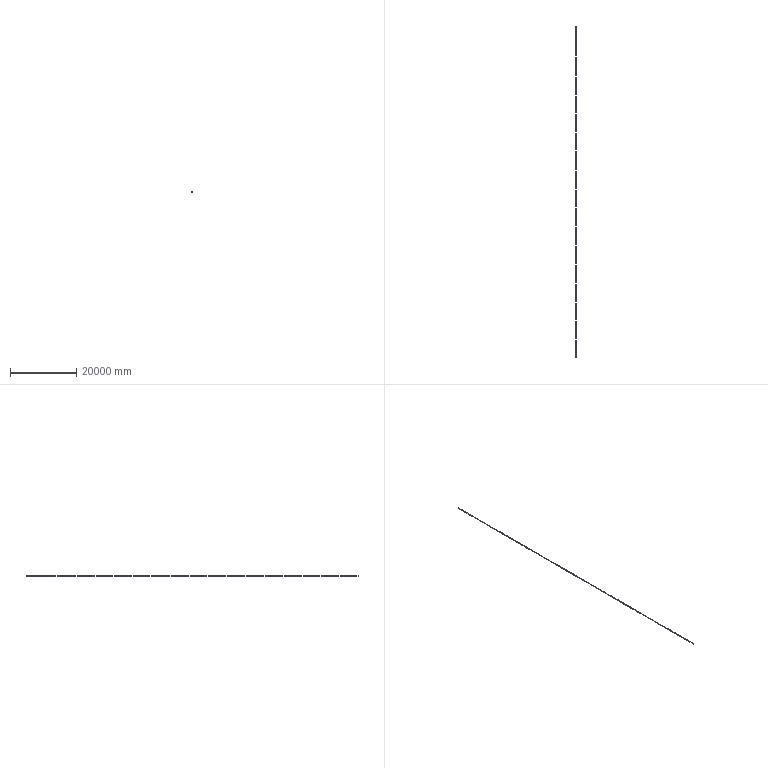Component | NX | DB1LIANJIE | 21 solids | 294 faces | volume 110114400 mm3 | plane 294